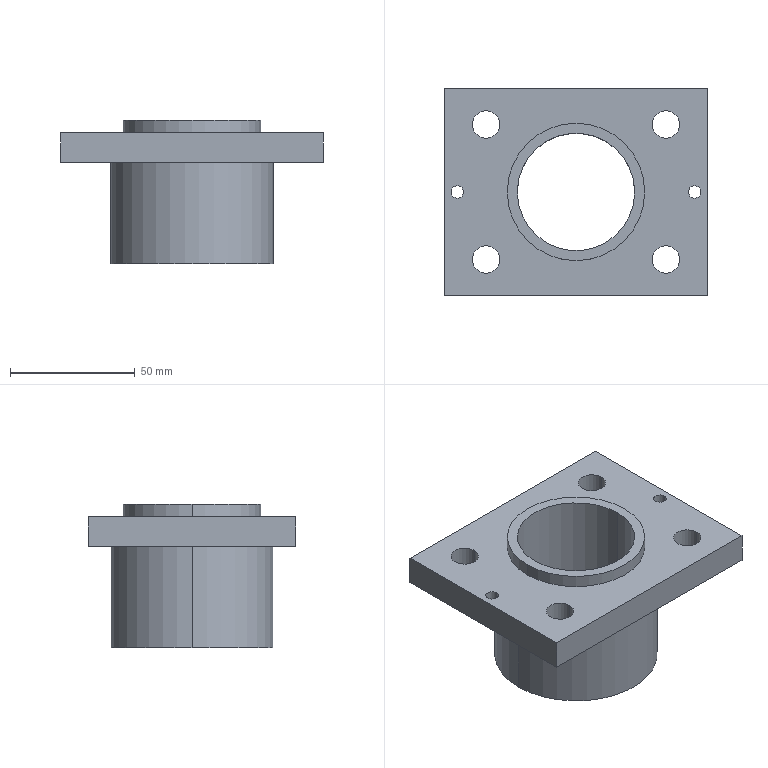Component | SolidWorks | 12AEncoderWheel-1_12AEncoderAxisRearBaffle-1 | 1 solid | 32 faces | box 105 x 83 x 57.5 mm | volume 145601 mm3 | cylinder 22 | plane 10 | commonest cylinder face diameters 11 x8 5 x4 47 x4 50 x2 55 x2 65 x2
build123d program:
from build123d import *

# Parameters (mm, degrees)
SKETCH1_W           = 83
SKETCH1_H           = 105
BOSS_EXTRUDE1_DEPTH = 12
SKETCH2_R           = 32.5
BOSS_EXTRUDE2_DEPTH = 57.5
SKETCH3_R           = 32.5
SKETCH3_R_2         = 27.5
CUT_EXTRUDE1_DEPTH  = 5
SKETCH4_R           = 23.5
CUT_EXTRUDE2_DEPTH  = 89.231
CUT_EXTRUDE5_REACH  = 87.057
SKETCH7_R           = 5.5
M6_TAPPED_HOLE1_D   = 5
SKETCH10_W          = 25
SKETCH10_H          = 2


with BuildPart() as part:
    # Sketch1 → Boss-Extrude1 (new body)
    with BuildSketch(Plane(origin=(0, 0, 0), x_dir=(1, 0, 0), z_dir=(0, 1, 0))):
        Rectangle(SKETCH1_W, SKETCH1_H)
    extrude(amount=BOSS_EXTRUDE1_DEPTH)

    # Sketch2 → Boss-Extrude2 (add)
    with BuildSketch(Plane.XZ.offset(5)):
        with Locations(Location((0, 0, 0), (0, 0, 270))):
            Circle(SKETCH2_R)
    extrude(amount=-BOSS_EXTRUDE2_DEPTH)

    # Sketch3 → Cut-Extrude1 (cut)
    with BuildSketch(Plane.XZ.offset(5)):
        with Locations(Location((0, 0, 0), (0, 0, 270))):
            Circle(SKETCH3_R)
        with Locations(Location((0, 0, 0), (0, 0, 270))):
            Circle(SKETCH3_R_2, mode=Mode.SUBTRACT)
    extrude(amount=-CUT_EXTRUDE1_DEPTH, mode=Mode.SUBTRACT)

    # Sketch4 → Cut-Extrude2 (cut, through all)
    with BuildSketch(Plane(origin=(0, 52.5, 0), x_dir=(1, 0, 0), z_dir=(0, 1, 0))):
        with Locations(Location((0, 0, 0), (0, 0, 270))):
            Circle(SKETCH4_R)
    extrude(amount=-CUT_EXTRUDE2_DEPTH, mode=Mode.SUBTRACT)

    # Sketch7 → Cut-Extrude5 (cut, up to next)
    with BuildSketch(Plane.XZ, mode=Mode.PRIVATE) as cut_extrude5_sk1:
        with Locations(Location((-27, 36, 0), (0, 0, 270))):
            Circle(SKETCH7_R)
    cut_extrude5_tool1 = extrude(cut_extrude5_sk1.sketch, amount=-CUT_EXTRUDE5_REACH, mode=Mode.PRIVATE) & part.part
    # Sketch7 → Cut-Extrude5 (cut, up to next)
    with BuildSketch(Plane.XZ, mode=Mode.PRIVATE) as cut_extrude5_sk2:
        with Locations(Location((27, 36, 0), (0, 0, 90))):
            Circle(SKETCH7_R)
    cut_extrude5_tool2 = extrude(cut_extrude5_sk2.sketch, amount=-CUT_EXTRUDE5_REACH, mode=Mode.PRIVATE) & part.part
    # Sketch7 → Cut-Extrude5 (cut, up to next)
    with BuildSketch(Plane.XZ, mode=Mode.PRIVATE) as cut_extrude5_sk3:
        with Locations(Location((27, -36, 0), (0, 0, 270))):
            Circle(SKETCH7_R)
    cut_extrude5_tool3 = extrude(cut_extrude5_sk3.sketch, amount=-CUT_EXTRUDE5_REACH, mode=Mode.PRIVATE) & part.part
    # Sketch7 → Cut-Extrude5 (cut, up to next)
    with BuildSketch(Plane.XZ, mode=Mode.PRIVATE) as cut_extrude5_sk4:
        with Locations(Location((-27, -36, 0), (0, 0, 90))):
            Circle(SKETCH7_R)
    cut_extrude5_tool4 = extrude(cut_extrude5_sk4.sketch, amount=-CUT_EXTRUDE5_REACH, mode=Mode.PRIVATE) & part.part
    add(cut_extrude5_tool1.solids().sort_by_distance((-27, 0, 36))[0], mode=Mode.SUBTRACT)
    add(cut_extrude5_tool2.solids().sort_by_distance((27, 0, 36))[0], mode=Mode.SUBTRACT)
    add(cut_extrude5_tool3.solids().sort_by_distance((27, 0, -36))[0], mode=Mode.SUBTRACT)
    add(cut_extrude5_tool4.solids().sort_by_distance((-27, 0, -36))[0], mode=Mode.SUBTRACT)

    # M6 Tapped Hole1 (through all)
    with Locations(Plane(origin=(0, 12, 0), x_dir=(1, 0, 0), z_dir=(0, 1, 0))):
        with Locations((0, 47.5), (0, -47.5)):
            Hole(M6_TAPPED_HOLE1_D / 2)

    # Sketch10 → Cut-Revolve1 (revolve, cut)
    with BuildSketch(Plane.XY, mode=Mode.PRIVATE) as cut_revolve1_sk:
        with Locations((12.5, 48.5)):
            Rectangle(SKETCH10_W, SKETCH10_H)
    revolve(cut_revolve1_sk.sketch.rotate(Axis((0, 0, 0), (0, 1, 0)), 270), axis=Axis((0, 0, 0), (0, 1, 0)), mode=Mode.SUBTRACT)


solid = part.part

# Placed as in the assembly
solid = solid.moved(Location((120.894, 147.181, -14.25), (-90, 90, 0)))
STEP:
#1=COLOUR_RGB('',0.7922,0.8196,0.9333);
#2=FILL_AREA_STYLE_COLOUR('',#1);
#3=FILL_AREA_STYLE('',(#2));
#4=SURFACE_STYLE_FILL_AREA(#3);
#5=SURFACE_SIDE_STYLE('',(#4));
#6=SURFACE_STYLE_USAGE(.BOTH.,#5);
#7=PRESENTATION_STYLE_ASSIGNMENT((#6));
#8=CARTESIAN_POINT('',(5.744,5.795,-2.51));
#9=VERTEX_POINT('',#8);
#10=CARTESIAN_POINT('',(3.775,5.795,-2.51));
#11=VERTEX_POINT('',#10);
#12=CARTESIAN_POINT('',(4.76,5.795,-2.51));
#13=DIRECTION('',(0.,0.,1.));
#14=DIRECTION('',(-1.,0.,0.));
#15=AXIS2_PLACEMENT_3D('',#12,#13,#14);
#16=CIRCLE('',#15,0.9843);
#17=EDGE_CURVE('',#9,#11,#16,.T.);
#18=ORIENTED_EDGE('',*,*,#17,.F.);
#19=CARTESIAN_POINT('',(5.744,5.795,-2.431));
#20=VERTEX_POINT('',#19);
#21=CARTESIAN_POINT('',(5.744,5.795,-0.561));
#22=DIRECTION('',(0.,0.,1.));
#23=VECTOR('',#22,39.37);
#24=LINE('',#21,#23);
#25=EDGE_CURVE('',#9,#20,#24,.T.);
#26=ORIENTED_EDGE('',*,*,#25,.T.);
#27=CARTESIAN_POINT('',(3.775,5.795,-2.431));
#28=VERTEX_POINT('',#27);
#29=CARTESIAN_POINT('',(4.76,5.795,-2.431));
#30=DIRECTION('',(0.,0.,1.));
#31=DIRECTION('',(-1.,0.,0.));
#32=AXIS2_PLACEMENT_3D('',#29,#30,#31);
#33=CIRCLE('',#32,0.9843);
#34=EDGE_CURVE('',#20,#28,#33,.T.);
#35=ORIENTED_EDGE('',*,*,#34,.T.);
#36=CARTESIAN_POINT('',(3.775,5.795,-0.561));
#37=DIRECTION('',(0.,0.,1.));
#38=VECTOR('',#37,39.37);
#39=LINE('',#36,#38);
#40=EDGE_CURVE('',#11,#28,#39,.T.);
#41=ORIENTED_EDGE('',*,*,#40,.F.);
#42=EDGE_LOOP('',(#18,#26,#35,#41));
#43=FACE_OUTER_BOUND('',#42,.T.);
#44=CARTESIAN_POINT('',(4.76,5.795,-0.561));
#45=DIRECTION('',(0.,0.,1.));
#46=DIRECTION('',(-1.,0.,0.));
#47=AXIS2_PLACEMENT_3D('',#44,#45,#46);
#48=CYLINDRICAL_SURFACE('',#47,0.9843);
#49=ADVANCED_FACE('',(#43),#48,.F.);
#50=CARTESIAN_POINT('',(2.791,5.795,-0.561));
#51=VERTEX_POINT('',#50);
#52=CARTESIAN_POINT('',(2.988,5.795,-0.561));
#53=VERTEX_POINT('',#52);
#54=CARTESIAN_POINT('',(2.89,5.795,-0.561));
#55=DIRECTION('',(-0.,-0.,-1.));
#56=DIRECTION('',(1.,0.,0.));
#57=AXIS2_PLACEMENT_3D('',#54,#55,#56);
#58=CIRCLE('',#57,0.09843);
#59=EDGE_CURVE('',#51,#53,#58,.T.);
#60=ORIENTED_EDGE('',*,*,#59,.F.);
#61=CARTESIAN_POINT('',(2.791,5.795,-1.033));
#62=VERTEX_POINT('',#61);
#63=CARTESIAN_POINT('',(2.791,5.795,-1.033));
#64=DIRECTION('',(-0.,-0.,-1.));
#65=VECTOR('',#64,39.37);
#66=LINE('',#63,#65);
#67=EDGE_CURVE('',#51,#62,#66,.T.);
#68=ORIENTED_EDGE('',*,*,#67,.T.);
#69=CARTESIAN_POINT('',(2.988,5.795,-1.033));
#70=VERTEX_POINT('',#69);
#71=CARTESIAN_POINT('',(2.89,5.795,-1.033));
#72=DIRECTION('',(-0.,-0.,-1.));
#73=DIRECTION('',(1.,0.,0.));
#74=AXIS2_PLACEMENT_3D('',#71,#72,#73);
#75=CIRCLE('',#74,0.09843);
#76=EDGE_CURVE('',#62,#70,#75,.T.);
#77=ORIENTED_EDGE('',*,*,#76,.T.);
#78=CARTESIAN_POINT('',(2.988,5.795,-1.033));
#79=DIRECTION('',(-0.,-0.,-1.));
#80=VECTOR('',#79,39.37);
#81=LINE('',#78,#80);
#82=EDGE_CURVE('',#53,#70,#81,.T.);
#83=ORIENTED_EDGE('',*,*,#82,.F.);
#84=EDGE_LOOP('',(#60,#68,#77,#83));
#85=FACE_OUTER_BOUND('',#84,.T.);
#86=CARTESIAN_POINT('',(2.89,5.795,-1.033));
#87=DIRECTION('',(-0.,-0.,-1.));
#88=DIRECTION('',(1.,0.,0.));
#89=AXIS2_PLACEMENT_3D('',#86,#87,#88);
#90=CYLINDRICAL_SURFACE('',#89,0.09843);
#91=ADVANCED_FACE('',(#85),#90,.F.);
#92=CARTESIAN_POINT('',(6.531,5.795,-0.561));
#93=VERTEX_POINT('',#92);
#94=CARTESIAN_POINT('',(6.728,5.795,-0.561));
#95=VERTEX_POINT('',#94);
#96=CARTESIAN_POINT('',(6.63,5.795,-0.561));
#97=DIRECTION('',(-0.,-0.,-1.));
#98=DIRECTION('',(1.,0.,0.));
#99=AXIS2_PLACEMENT_3D('',#96,#97,#98);
#100=CIRCLE('',#99,0.09843);
#101=EDGE_CURVE('',#93,#95,#100,.T.);
#102=ORIENTED_EDGE('',*,*,#101,.F.);
#103=CARTESIAN_POINT('',(6.531,5.795,-1.033));
#104=VERTEX_POINT('',#103);
#105=CARTESIAN_POINT('',(6.531,5.795,-1.033));
#106=DIRECTION('',(-0.,-0.,-1.));
#107=VECTOR('',#106,39.37);
#108=LINE('',#105,#107);
#109=EDGE_CURVE('',#93,#104,#108,.T.);
#110=ORIENTED_EDGE('',*,*,#109,.T.);
#111=CARTESIAN_POINT('',(6.728,5.795,-1.033));
#112=VERTEX_POINT('',#111);
#113=CARTESIAN_POINT('',(6.63,5.795,-1.033));
#114=DIRECTION('',(-0.,-0.,-1.));
#115=DIRECTION('',(1.,0.,0.));
#116=AXIS2_PLACEMENT_3D('',#113,#114,#115);
#117=CIRCLE('',#116,0.09843);
#118=EDGE_CURVE('',#104,#112,#117,.T.);
#119=ORIENTED_EDGE('',*,*,#118,.T.);
#120=CARTESIAN_POINT('',(6.728,5.795,-1.033));
#121=DIRECTION('',(-0.,-0.,-1.));
#122=VECTOR('',#121,39.37);
#123=LINE('',#120,#122);
#124=EDGE_CURVE('',#95,#112,#123,.T.);
#125=ORIENTED_EDGE('',*,*,#124,.F.);
#126=EDGE_LOOP('',(#102,#110,#119,#125));
#127=FACE_OUTER_BOUND('',#126,.T.);
#128=CARTESIAN_POINT('',(6.63,5.795,-1.033));
#129=DIRECTION('',(-0.,-0.,-1.));
#130=DIRECTION('',(1.,0.,0.));
#131=AXIS2_PLACEMENT_3D('',#128,#129,#130);
#132=CYLINDRICAL_SURFACE('',#131,0.09843);
#133=ADVANCED_FACE('',(#127),#132,.F.);
#134=CARTESIAN_POINT('',(3.559,6.858,-1.033));
#135=VERTEX_POINT('',#134);
#136=CARTESIAN_POINT('',(3.126,6.858,-1.033));
#137=VERTEX_POINT('',#136);
#138=CARTESIAN_POINT('',(3.342,6.858,-1.033));
#139=DIRECTION('',(0.,0.,1.));
#140=DIRECTION('',(1.,0.,0.));
#141=AXIS2_PLACEMENT_3D('',#138,#139,#140);
#142=CIRCLE('',#141,0.2165);
#143=EDGE_CURVE('',#135,#137,#142,.T.);
#144=ORIENTED_EDGE('',*,*,#143,.F.);
#145=CARTESIAN_POINT('',(3.559,6.858,-0.561));
#146=VERTEX_POINT('',#145);
#147=CARTESIAN_POINT('',(3.559,6.858,-2.628));
#148=DIRECTION('',(0.,0.,1.));
#149=VECTOR('',#148,39.37);
#150=LINE('',#147,#149);
#151=EDGE_CURVE('',#135,#146,#150,.T.);
#152=ORIENTED_EDGE('',*,*,#151,.T.);
#153=CARTESIAN_POINT('',(3.126,6.858,-0.561));
#154=VERTEX_POINT('',#153);
#155=CARTESIAN_POINT('',(3.342,6.858,-0.561));
#156=DIRECTION('',(0.,0.,1.));
#157=DIRECTION('',(1.,0.,0.));
#158=AXIS2_PLACEMENT_3D('',#155,#156,#157);
#159=CIRCLE('',#158,0.2165);
#160=EDGE_CURVE('',#146,#154,#159,.T.);
#161=ORIENTED_EDGE('',*,*,#160,.T.);
#162=CARTESIAN_POINT('',(3.126,6.858,-2.628));
#163=DIRECTION('',(0.,0.,1.));
#164=VECTOR('',#163,39.37);
#165=LINE('',#162,#164);
#166=EDGE_CURVE('',#137,#154,#165,.T.);
#167=ORIENTED_EDGE('',*,*,#166,.F.);
#168=EDGE_LOOP('',(#144,#152,#161,#167));
#169=FACE_OUTER_BOUND('',#168,.T.);
#170=CARTESIAN_POINT('',(3.342,6.858,-2.628));
#171=DIRECTION('',(0.,0.,1.));
#172=DIRECTION('',(-1.,0.,0.));
#173=AXIS2_PLACEMENT_3D('',#170,#171,#172);
#174=CYLINDRICAL_SURFACE('',#173,0.2165);
#175=ADVANCED_FACE('',(#169),#174,.F.);
#176=CARTESIAN_POINT('',(3.559,4.732,-1.033));
#177=VERTEX_POINT('',#176);
#178=CARTESIAN_POINT('',(3.126,4.732,-1.033));
#179=VERTEX_POINT('',#178);
#180=CARTESIAN_POINT('',(3.342,4.732,-1.033));
#181=DIRECTION('',(0.,0.,1.));
#182=DIRECTION('',(1.,0.,0.));
#183=AXIS2_PLACEMENT_3D('',#180,#181,#182);
#184=CIRCLE('',#183,0.2165);
#185=EDGE_CURVE('',#177,#179,#184,.T.);
#186=ORIENTED_EDGE('',*,*,#185,.F.);
#187=CARTESIAN_POINT('',(3.559,4.732,-0.561));
#188=VERTEX_POINT('',#187);
#189=CARTESIAN_POINT('',(3.559,4.732,-2.628));
#190=DIRECTION('',(0.,0.,1.));
#191=VECTOR('',#190,39.37);
#192=LINE('',#189,#191);
#193=EDGE_CURVE('',#177,#188,#192,.T.);
#194=ORIENTED_EDGE('',*,*,#193,.T.);
#195=CARTESIAN_POINT('',(3.126,4.732,-0.561));
#196=VERTEX_POINT('',#195);
#197=CARTESIAN_POINT('',(3.342,4.732,-0.561));
#198=DIRECTION('',(0.,0.,1.));
#199=DIRECTION('',(-1.,0.,0.));
#200=AXIS2_PLACEMENT_3D('',#197,#198,#199);
#201=CIRCLE('',#200,0.2165);
#202=EDGE_CURVE('',#188,#196,#201,.T.);
#203=ORIENTED_EDGE('',*,*,#202,.T.);
#204=CARTESIAN_POINT('',(3.126,4.732,-2.628));
#205=DIRECTION('',(0.,0.,1.));
#206=VECTOR('',#205,39.37);
#207=LINE('',#204,#206);
#208=EDGE_CURVE('',#179,#196,#207,.T.);
#209=ORIENTED_EDGE('',*,*,#208,.F.);
#210=EDGE_LOOP('',(#186,#194,#203,#209));
#211=FACE_OUTER_BOUND('',#210,.T.);
#212=CARTESIAN_POINT('',(3.342,4.732,-2.628));
#213=DIRECTION('',(0.,0.,1.));
#214=DIRECTION('',(-1.,0.,0.));
#215=AXIS2_PLACEMENT_3D('',#212,#213,#214);
#216=CYLINDRICAL_SURFACE('',#215,0.2165);
#217=ADVANCED_FACE('',(#211),#216,.F.);
#218=CARTESIAN_POINT('',(6.393,4.732,-1.033));
#219=VERTEX_POINT('',#218);
#220=CARTESIAN_POINT('',(5.96,4.732,-1.033));
#221=VERTEX_POINT('',#220);
#222=CARTESIAN_POINT('',(6.177,4.732,-1.033));
#223=DIRECTION('',(0.,0.,1.));
#224=DIRECTION('',(1.,0.,0.));
#225=AXIS2_PLACEMENT_3D('',#222,#223,#224);
#226=CIRCLE('',#225,0.2165);
#227=EDGE_CURVE('',#219,#221,#226,.T.);
#228=ORIENTED_EDGE('',*,*,#227,.F.);
#229=CARTESIAN_POINT('',(6.393,4.732,-0.561));
#230=VERTEX_POINT('',#229);
#231=CARTESIAN_POINT('',(6.393,4.732,-2.628));
#232=DIRECTION('',(0.,0.,1.));
#233=VECTOR('',#232,39.37);
#234=LINE('',#231,#233);
#235=EDGE_CURVE('',#219,#230,#234,.T.);
#236=ORIENTED_EDGE('',*,*,#235,.T.);
#237=CARTESIAN_POINT('',(5.96,4.732,-0.561));
#238=VERTEX_POINT('',#237);
#239=CARTESIAN_POINT('',(6.177,4.732,-0.561));
#240=DIRECTION('',(0.,0.,1.));
#241=DIRECTION('',(1.,0.,0.));
#242=AXIS2_PLACEMENT_3D('',#239,#240,#241);
#243=CIRCLE('',#242,0.2165);
#244=EDGE_CURVE('',#230,#238,#243,.T.);
#245=ORIENTED_EDGE('',*,*,#244,.T.);
#246=CARTESIAN_POINT('',(5.96,4.732,-2.628));
#247=DIRECTION('',(0.,0.,1.));
#248=VECTOR('',#247,39.37);
#249=LINE('',#246,#248);
#250=EDGE_CURVE('',#221,#238,#249,.T.);
#251=ORIENTED_EDGE('',*,*,#250,.F.);
#252=EDGE_LOOP('',(#228,#236,#245,#251));
#253=FACE_OUTER_BOUND('',#252,.T.);
#254=CARTESIAN_POINT('',(6.177,4.732,-2.628));
#255=DIRECTION('',(0.,0.,1.));
#256=DIRECTION('',(-1.,0.,0.));
#257=AXIS2_PLACEMENT_3D('',#254,#255,#256);
#258=CYLINDRICAL_SURFACE('',#257,0.2165);
#259=ADVANCED_FACE('',(#253),#258,.F.);
#260=CARTESIAN_POINT('',(6.393,6.858,-1.033));
#261=VERTEX_POINT('',#260);
#262=CARTESIAN_POINT('',(5.96,6.858,-1.033));
#263=VERTEX_POINT('',#262);
#264=CARTESIAN_POINT('',(6.177,6.858,-1.033));
#265=DIRECTION('',(0.,0.,1.));
#266=DIRECTION('',(1.,0.,0.));
#267=AXIS2_PLACEMENT_3D('',#264,#265,#266);
#268=CIRCLE('',#267,0.2165);
#269=EDGE_CURVE('',#261,#263,#268,.T.);
#270=ORIENTED_EDGE('',*,*,#269,.F.);
#271=CARTESIAN_POINT('',(6.393,6.858,-0.561));
#272=VERTEX_POINT('',#271);
#273=CARTESIAN_POINT('',(6.393,6.858,-2.628));
#274=DIRECTION('',(0.,0.,1.));
#275=VECTOR('',#274,39.37);
#276=LINE('',#273,#275);
#277=EDGE_CURVE('',#261,#272,#276,.T.);
#278=ORIENTED_EDGE('',*,*,#277,.T.);
#279=CARTESIAN_POINT('',(5.96,6.858,-0.561));
#280=VERTEX_POINT('',#279);
#281=CARTESIAN_POINT('',(6.177,6.858,-0.561));
#282=DIRECTION('',(0.,0.,1.));
#283=DIRECTION('',(-1.,0.,0.));
#284=AXIS2_PLACEMENT_3D('',#281,#282,#283);
#285=CIRCLE('',#284,0.2165);
#286=EDGE_CURVE('',#272,#280,#285,.T.);
#287=ORIENTED_EDGE('',*,*,#286,.T.);
#288=CARTESIAN_POINT('',(5.96,6.858,-2.628));
#289=DIRECTION('',(0.,0.,1.));
#290=VECTOR('',#289,39.37);
#291=LINE('',#288,#290);
#292=EDGE_CURVE('',#263,#280,#291,.T.);
#293=ORIENTED_EDGE('',*,*,#292,.F.);
#294=EDGE_LOOP('',(#270,#278,#287,#293));
#295=FACE_OUTER_BOUND('',#294,.T.);
#296=CARTESIAN_POINT('',(6.177,6.858,-2.628));
#297=DIRECTION('',(0.,0.,1.));
#298=DIRECTION('',(-1.,0.,0.));
#299=AXIS2_PLACEMENT_3D('',#296,#297,#298);
#300=CYLINDRICAL_SURFACE('',#299,0.2165);
#301=ADVANCED_FACE('',(#295),#300,.F.);
#302=CARTESIAN_POINT('',(3.834,5.795,-0.3642));
#303=VERTEX_POINT('',#302);
#304=CARTESIAN_POINT('',(5.685,5.795,-0.3642));
#305=VERTEX_POINT('',#304);
#306=CARTESIAN_POINT('',(4.76,5.795,-0.3642));
#307=DIRECTION('',(-0.,-0.,-1.));
#308=DIRECTION('',(1.,0.,0.));
#309=AXIS2_PLACEMENT_3D('',#306,#307,#308);
#310=CIRCLE('',#309,0.9252);
#311=EDGE_CURVE('',#303,#305,#310,.T.);
#312=ORIENTED_EDGE('',*,*,#311,.F.);
#313=CARTESIAN_POINT('',(3.834,5.795,-2.431));
#314=VERTEX_POINT('',#313);
#315=CARTESIAN_POINT('',(3.834,5.795,-0.3642));
#316=DIRECTION('',(-0.,-0.,-1.));
#317=VECTOR('',#316,39.37);
#318=LINE('',#315,#317);
#319=EDGE_CURVE('',#303,#314,#318,.T.);
#320=ORIENTED_EDGE('',*,*,#319,.T.);
#321=CARTESIAN_POINT('',(5.685,5.795,-2.431));
#322=VERTEX_POINT('',#321);
#323=CARTESIAN_POINT('',(4.76,5.795,-2.431));
#324=DIRECTION('',(-0.,-0.,-1.));
#325=DIRECTION('',(-1.,0.,0.));
#326=AXIS2_PLACEMENT_3D('',#323,#324,#325);
#327=CIRCLE('',#326,0.9252);
#328=EDGE_CURVE('',#314,#322,#327,.T.);
#329=ORIENTED_EDGE('',*,*,#328,.T.);
#330=CARTESIAN_POINT('',(5.685,5.795,-0.3642));
#331=DIRECTION('',(-0.,-0.,-1.));
#332=VECTOR('',#331,39.37);
#333=LINE('',#330,#332);
#334=EDGE_CURVE('',#305,#322,#333,.T.);
#335=ORIENTED_EDGE('',*,*,#334,.F.);
#336=EDGE_LOOP('',(#312,#320,#329,#335));
#337=FACE_OUTER_BOUND('',#336,.T.);
#338=CARTESIAN_POINT('',(4.76,5.795,-0.3642));
#339=DIRECTION('',(-0.,-0.,-1.));
#340=DIRECTION('',(1.,0.,0.));
#341=AXIS2_PLACEMENT_3D('',#338,#339,#340);
#342=CYLINDRICAL_SURFACE('',#341,0.9252);
#343=ADVANCED_FACE('',(#337),#342,.F.);
#344=CARTESIAN_POINT('',(3.677,5.795,-0.561));
#345=VERTEX_POINT('',#344);
#346=CARTESIAN_POINT('',(5.842,5.795,-0.561));
#347=VERTEX_POINT('',#346);
#348=CARTESIAN_POINT('',(4.76,5.795,-0.561));
#349=DIRECTION('',(0.,0.,1.));
#350=DIRECTION('',(-1.,0.,0.));
#351=AXIS2_PLACEMENT_3D('',#348,#349,#350);
#352=CIRCLE('',#351,1.083);
#353=EDGE_CURVE('',#345,#347,#352,.T.);
#354=ORIENTED_EDGE('',*,*,#353,.T.);
#355=CARTESIAN_POINT('',(5.842,5.795,-0.3642));
#356=VERTEX_POINT('',#355);
#357=CARTESIAN_POINT('',(5.842,5.795,-0.561));
#358=DIRECTION('',(0.,0.,1.));
#359=VECTOR('',#358,39.37);
#360=LINE('',#357,#359);
#361=EDGE_CURVE('',#347,#356,#360,.T.);
#362=ORIENTED_EDGE('',*,*,#361,.T.);
#363=CARTESIAN_POINT('',(3.677,5.795,-0.3642));
#364=VERTEX_POINT('',#363);
#365=CARTESIAN_POINT('',(4.76,5.795,-0.3642));
#366=DIRECTION('',(0.,0.,1.));
#367=DIRECTION('',(-1.,0.,0.));
#368=AXIS2_PLACEMENT_3D('',#365,#366,#367);
#369=CIRCLE('',#368,1.083);
#370=EDGE_CURVE('',#364,#356,#369,.T.);
#371=ORIENTED_EDGE('',*,*,#370,.F.);
#372=CARTESIAN_POINT('',(3.677,5.795,-0.561));
#373=DIRECTION('',(0.,0.,1.));
#374=VECTOR('',#373,39.37);
#375=LINE('',#372,#374);
#376=EDGE_CURVE('',#345,#364,#375,.T.);
#377=ORIENTED_EDGE('',*,*,#376,.F.);
#378=EDGE_LOOP('',(#354,#362,#371,#377));
#379=FACE_OUTER_BOUND('',#378,.T.);
#380=CARTESIAN_POINT('',(4.76,5.795,-0.561));
#381=DIRECTION('',(0.,0.,1.));
#382=DIRECTION('',(-1.,0.,0.));
#383=AXIS2_PLACEMENT_3D('',#380,#381,#382);
#384=CYLINDRICAL_SURFACE('',#383,1.083);
#385=ADVANCED_FACE('',(#379),#384,.T.);
#386=CARTESIAN_POINT('',(3.48,5.795,-2.628));
#387=VERTEX_POINT('',#386);
#388=CARTESIAN_POINT('',(6.039,5.795,-2.628));
#389=VERTEX_POINT('',#388);
#390=CARTESIAN_POINT('',(4.76,5.795,-2.628));
#391=DIRECTION('',(0.,0.,1.));
#392=DIRECTION('',(-1.,0.,0.));
#393=AXIS2_PLACEMENT_3D('',#390,#391,#392);
#394=CIRCLE('',#393,1.28);
#395=EDGE_CURVE('',#387,#389,#394,.T.);
#396=ORIENTED_EDGE('',*,*,#395,.T.);
#397=CARTESIAN_POINT('',(6.039,5.795,-1.033));
#398=VERTEX_POINT('',#397);
#399=CARTESIAN_POINT('',(6.039,5.795,-2.628));
#400=DIRECTION('',(0.,0.,1.));
#401=VECTOR('',#400,39.37);
#402=LINE('',#399,#401);
#403=EDGE_CURVE('',#389,#398,#402,.T.);
#404=ORIENTED_EDGE('',*,*,#403,.T.);
#405=CARTESIAN_POINT('',(3.48,5.795,-1.033));
#406=VERTEX_POINT('',#405);
#407=CARTESIAN_POINT('',(4.76,5.795,-1.033));
#408=DIRECTION('',(-0.,-0.,-1.));
#409=DIRECTION('',(1.,0.,0.));
#410=AXIS2_PLACEMENT_3D('',#407,#408,#409);
#411=CIRCLE('',#410,1.28);
#412=EDGE_CURVE('',#398,#406,#411,.T.);
#413=ORIENTED_EDGE('',*,*,#412,.T.);
#414=CARTESIAN_POINT('',(3.48,5.795,-2.628));
#415=DIRECTION('',(0.,0.,1.));
#416=VECTOR('',#415,39.37);
#417=LINE('',#414,#416);
#418=EDGE_CURVE('',#387,#406,#417,.T.);
#419=ORIENTED_EDGE('',*,*,#418,.F.);
#420=EDGE_LOOP('',(#396,#404,#413,#419));
#421=FACE_OUTER_BOUND('',#420,.T.);
#422=CARTESIAN_POINT('',(4.76,5.795,-2.628));
#423=DIRECTION('',(0.,0.,1.));
#424=DIRECTION('',(-1.,0.,0.));
#425=AXIS2_PLACEMENT_3D('',#422,#423,#424);
#426=CYLINDRICAL_SURFACE('',#425,1.28);
#427=ADVANCED_FACE('',(#421),#426,.T.);
#428=CARTESIAN_POINT('',(5.685,5.795,-2.51));
#429=VERTEX_POINT('',#428);
#430=CARTESIAN_POINT('',(3.834,5.795,-2.51));
#431=VERTEX_POINT('',#430);
#432=CARTESIAN_POINT('',(4.76,5.795,-2.51));
#433=DIRECTION('',(0.,0.,1.));
#434=DIRECTION('',(1.,0.,0.));
#435=AXIS2_PLACEMENT_3D('',#432,#433,#434);
#436=CIRCLE('',#435,0.9252);
#437=EDGE_CURVE('',#429,#431,#436,.T.);
#438=ORIENTED_EDGE('',*,*,#437,.T.);
#439=CARTESIAN_POINT('',(3.834,5.795,-2.628));
#440=VERTEX_POINT('',#439);
#441=CARTESIAN_POINT('',(3.834,5.795,-0.3642));
#442=DIRECTION('',(-0.,-0.,-1.));
#443=VECTOR('',#442,39.37);
#444=LINE('',#441,#443);
#445=EDGE_CURVE('',#431,#440,#444,.T.);
#446=ORIENTED_EDGE('',*,*,#445,.T.);
#447=CARTESIAN_POINT('',(5.685,5.795,-2.628));
#448=VERTEX_POINT('',#447);
#449=CARTESIAN_POINT('',(4.76,5.795,-2.628));
#450=DIRECTION('',(-0.,-0.,-1.));
#451=DIRECTION('',(1.,0.,0.));
#452=AXIS2_PLACEMENT_3D('',#449,#450,#451);
#453=CIRCLE('',#452,0.9252);
#454=EDGE_CURVE('',#440,#448,#453,.T.);
#455=ORIENTED_EDGE('',*,*,#454,.T.);
#456=CARTESIAN_POINT('',(5.685,5.795,-0.3642));
#457=DIRECTION('',(-0.,-0.,-1.));
#458=VECTOR('',#457,39.37);
#459=LINE('',#456,#458);
#460=EDGE_CURVE('',#429,#448,#459,.T.);
#461=ORIENTED_EDGE('',*,*,#460,.F.);
#462=EDGE_LOOP('',(#438,#446,#455,#461));
#463=FACE_OUTER_BOUND('',#462,.T.);
#464=CARTESIAN_POINT('',(4.76,5.795,-0.3642));
#465=DIRECTION('',(-0.,-0.,-1.));
#466=DIRECTION('',(1.,0.,0.));
#467=AXIS2_PLACEMENT_3D('',#464,#465,#466);
#468=CYLINDRICAL_SURFACE('',#467,0.9252);
#469=ADVANCED_FACE('',(#463),#468,.F.);
#470=ORIENTED_EDGE('',*,*,#445,.F.);
#471=CARTESIAN_POINT('',(4.76,5.795,-2.51));
#472=DIRECTION('',(0.,0.,1.));
#473=DIRECTION('',(1.,0.,0.));
#474=AXIS2_PLACEMENT_3D('',#471,#472,#473);
#475=CIRCLE('',#474,0.9252);
#476=EDGE_CURVE('',#431,#429,#475,.T.);
#477=ORIENTED_EDGE('',*,*,#476,.T.);
#478=ORIENTED_EDGE('',*,*,#460,.T.);
#479=CARTESIAN_POINT('',(4.76,5.795,-2.628));
#480=DIRECTION('',(-0.,-0.,-1.));
#481=DIRECTION('',(1.,0.,0.));
#482=AXIS2_PLACEMENT_3D('',#479,#480,#481);
#483=CIRCLE('',#482,0.9252);
#484=EDGE_CURVE('',#448,#440,#483,.T.);
#485=ORIENTED_EDGE('',*,*,#484,.T.);
#486=EDGE_LOOP('',(#470,#477,#478,#485));
#487=FACE_OUTER_BOUND('',#486,.T.);
#488=CARTESIAN_POINT('',(4.76,5.795,-0.3642));
#489=DIRECTION('',(-0.,-0.,-1.));
#490=DIRECTION('',(1.,0.,0.));
#491=AXIS2_PLACEMENT_3D('',#488,#489,#490);
#492=CYLINDRICAL_SURFACE('',#491,0.9252);
#493=ADVANCED_FACE('',(#487),#492,.F.);
#494=CARTESIAN_POINT('',(6.827,4.161,-0.561));
#495=VERTEX_POINT('',#494);
#496=CARTESIAN_POINT('',(2.693,4.161,-0.561));
#497=VERTEX_POINT('',#496);
#498=CARTESIAN_POINT('',(2.693,4.161,-0.561));
#499=DIRECTION('',(-1.,-0.,0.));
#500=VECTOR('',#499,39.37);
#501=LINE('',#498,#500);
#502=EDGE_CURVE('',#495,#497,#501,.T.);
#503=ORIENTED_EDGE('',*,*,#502,.T.);
#504=CARTESIAN_POINT('',(2.693,4.161,-1.033));
#505=VERTEX_POINT('',#504);
#506=CARTESIAN_POINT('',(2.693,4.161,-1.033));
#507=DIRECTION('',(0.,0.,1.));
#508=VECTOR('',#507,39.37);
#509=LINE('',#506,#508);
#510=EDGE_CURVE('',#505,#497,#509,.T.);
#511=ORIENTED_EDGE('',*,*,#510,.F.);
#512=CARTESIAN_POINT('',(6.827,4.161,-1.033));
#513=VERTEX_POINT('',#512);
#514=CARTESIAN_POINT('',(2.693,4.161,-1.033));
#515=DIRECTION('',(-1.,-0.,0.));
#516=VECTOR('',#515,39.37);
#517=LINE('',#514,#516);
#518=EDGE_CURVE('',#513,#505,#517,.T.);
#519=ORIENTED_EDGE('',*,*,#518,.F.);
#520=CARTESIAN_POINT('',(6.827,4.161,-1.033));
#521=DIRECTION('',(0.,0.,1.));
#522=VECTOR('',#521,39.37);
#523=LINE('',#520,#522);
#524=EDGE_CURVE('',#513,#495,#523,.T.);
#525=ORIENTED_EDGE('',*,*,#524,.T.);
#526=EDGE_LOOP('',(#503,#511,#519,#525));
#527=FACE_OUTER_BOUND('',#526,.T.);
#528=CARTESIAN_POINT('',(2.693,4.161,-1.033));
#529=DIRECTION('',(-0.,1.,-0.));
#530=DIRECTION('',(1.,0.,-0.));
#531=AXIS2_PLACEMENT_3D('',#528,#529,#530);
#532=PLANE('',#531);
#533=ADVANCED_FACE('',(#527),#532,.F.);
#534=CARTESIAN_POINT('',(2.693,7.428,-0.561));
#535=VERTEX_POINT('',#534);
#536=CARTESIAN_POINT('',(2.693,7.428,-0.561));
#537=DIRECTION('',(-0.,1.,-0.));
#538=VECTOR('',#537,39.37);
#539=LINE('',#536,#538);
#540=EDGE_CURVE('',#497,#535,#539,.T.);
#541=ORIENTED_EDGE('',*,*,#540,.T.);
#542=CARTESIAN_POINT('',(2.693,7.428,-1.033));
#543=VERTEX_POINT('',#542);
#544=CARTESIAN_POINT('',(2.693,7.428,-1.033));
#545=DIRECTION('',(0.,0.,1.));
#546=VECTOR('',#545,39.37);
#547=LINE('',#544,#546);
#548=EDGE_CURVE('',#543,#535,#547,.T.);
#549=ORIENTED_EDGE('',*,*,#548,.F.);
#550=CARTESIAN_POINT('',(2.693,7.428,-1.033));
#551=DIRECTION('',(-0.,1.,-0.));
#552=VECTOR('',#551,39.37);
#553=LINE('',#550,#552);
#554=EDGE_CURVE('',#505,#543,#553,.T.);
#555=ORIENTED_EDGE('',*,*,#554,.F.);
#556=ORIENTED_EDGE('',*,*,#510,.T.);
#557=EDGE_LOOP('',(#541,#549,#555,#556));
#558=FACE_OUTER_BOUND('',#557,.T.);
#559=CARTESIAN_POINT('',(2.693,7.428,-1.033));
#560=DIRECTION('',(1.,0.,-0.));
#561=DIRECTION('',(0.,-1.,0.));
#562=AXIS2_PLACEMENT_3D('',#559,#560,#561);
#563=PLANE('',#562);
#564=ADVANCED_FACE('',(#558),#563,.F.);
#565=CARTESIAN_POINT('',(6.827,7.428,-0.561));
#566=VERTEX_POINT('',#565);
#567=CARTESIAN_POINT('',(2.693,7.428,-0.561));
#568=DIRECTION('',(1.,0.,-0.));
#569=VECTOR('',#568,39.37);
#570=LINE('',#567,#569);
#571=EDGE_CURVE('',#535,#566,#570,.T.);
#572=ORIENTED_EDGE('',*,*,#571,.T.);
#573=CARTESIAN_POINT('',(6.827,7.428,-1.033));
#574=VERTEX_POINT('',#573);
#575=CARTESIAN_POINT('',(6.827,7.428,-1.033));
#576=DIRECTION('',(0.,0.,1.));
#577=VECTOR('',#576,39.37);
#578=LINE('',#575,#577);
#579=EDGE_CURVE('',#574,#566,#578,.T.);
#580=ORIENTED_EDGE('',*,*,#579,.F.);
#581=CARTESIAN_POINT('',(2.693,7.428,-1.033));
#582=DIRECTION('',(1.,0.,-0.));
#583=VECTOR('',#582,39.37);
#584=LINE('',#581,#583);
#585=EDGE_CURVE('',#543,#574,#584,.T.);
#586=ORIENTED_EDGE('',*,*,#585,.F.);
#587=ORIENTED_EDGE('',*,*,#548,.T.);
#588=EDGE_LOOP('',(#572,#580,#586,#587));
#589=FACE_OUTER_BOUND('',#588,.T.);
#590=CARTESIAN_POINT('',(2.693,7.428,-1.033));
#591=DIRECTION('',(0.,-1.,0.));
#592=DIRECTION('',(-1.,-0.,0.));
#593=AXIS2_PLACEMENT_3D('',#590,#591,#592);
#594=PLANE('',#593);
#595=ADVANCED_FACE('',(#589),#594,.F.);
#596=CARTESIAN_POINT('',(6.827,7.428,-0.561));
#597=DIRECTION('',(0.,-1.,0.));
#598=VECTOR('',#597,39.37);
#599=LINE('',#596,#598);
#600=EDGE_CURVE('',#566,#495,#599,.T.);
#601=ORIENTED_EDGE('',*,*,#600,.T.);
#602=ORIENTED_EDGE('',*,*,#524,.F.);
#603=CARTESIAN_POINT('',(6.827,7.428,-1.033));
#604=DIRECTION('',(0.,-1.,0.));
#605=VECTOR('',#604,39.37);
#606=LINE('',#603,#605);
#607=EDGE_CURVE('',#574,#513,#606,.T.);
#608=ORIENTED_EDGE('',*,*,#607,.F.);
#609=ORIENTED_EDGE('',*,*,#579,.T.);
#610=EDGE_LOOP('',(#601,#602,#608,#609));
#611=FACE_OUTER_BOUND('',#610,.T.);
#612=CARTESIAN_POINT('',(6.827,7.428,-1.033));
#613=DIRECTION('',(-1.,-0.,0.));
#614=DIRECTION('',(-0.,1.,-0.));
#615=AXIS2_PLACEMENT_3D('',#612,#613,#614);
#616=PLANE('',#615);
#617=ADVANCED_FACE('',(#611),#616,.F.);
#618=CARTESIAN_POINT('',(2.89,5.795,-1.033));
#619=DIRECTION('',(-0.,-0.,-1.));
#620=DIRECTION('',(1.,0.,0.));
#621=AXIS2_PLACEMENT_3D('',#618,#619,#620);
#622=CIRCLE('',#621,0.09843);
#623=EDGE_CURVE('',#70,#62,#622,.T.);
#624=ORIENTED_EDGE('',*,*,#623,.F.);
#625=ORIENTED_EDGE('',*,*,#76,.F.);
#626=EDGE_LOOP('',(#624,#625));
#627=FACE_BOUND('',#626,.T.);
#628=CARTESIAN_POINT('',(6.63,5.795,-1.033));
#629=DIRECTION('',(-0.,-0.,-1.));
#630=DIRECTION('',(1.,0.,0.));
#631=AXIS2_PLACEMENT_3D('',#628,#629,#630);
#632=CIRCLE('',#631,0.09843);
#633=EDGE_CURVE('',#112,#104,#632,.T.);
#634=ORIENTED_EDGE('',*,*,#633,.F.);
#635=ORIENTED_EDGE('',*,*,#118,.F.);
#636=EDGE_LOOP('',(#634,#635));
#637=FACE_BOUND('',#636,.T.);
#638=CARTESIAN_POINT('',(3.342,6.858,-1.033));
#639=DIRECTION('',(0.,0.,1.));
#640=DIRECTION('',(1.,0.,0.));
#641=AXIS2_PLACEMENT_3D('',#638,#639,#640);
#642=CIRCLE('',#641,0.2165);
#643=EDGE_CURVE('',#137,#135,#642,.T.);
#644=ORIENTED_EDGE('',*,*,#643,.T.);
#645=ORIENTED_EDGE('',*,*,#143,.T.);
#646=EDGE_LOOP('',(#644,#645));
#647=FACE_BOUND('',#646,.T.);
#648=CARTESIAN_POINT('',(3.342,4.732,-1.033));
#649=DIRECTION('',(0.,0.,1.));
#650=DIRECTION('',(1.,0.,0.));
#651=AXIS2_PLACEMENT_3D('',#648,#649,#650);
#652=CIRCLE('',#651,0.2165);
#653=EDGE_CURVE('',#179,#177,#652,.T.);
#654=ORIENTED_EDGE('',*,*,#653,.T.);
#655=ORIENTED_EDGE('',*,*,#185,.T.);
#656=EDGE_LOOP('',(#654,#655));
#657=FACE_BOUND('',#656,.T.);
#658=CARTESIAN_POINT('',(6.177,4.732,-1.033));
#659=DIRECTION('',(0.,0.,1.));
#660=DIRECTION('',(1.,0.,0.));
#661=AXIS2_PLACEMENT_3D('',#658,#659,#660);
#662=CIRCLE('',#661,0.2165);
#663=EDGE_CURVE('',#221,#219,#662,.T.);
#664=ORIENTED_EDGE('',*,*,#663,.T.);
#665=ORIENTED_EDGE('',*,*,#227,.T.);
#666=EDGE_LOOP('',(#664,#665));
#667=FACE_BOUND('',#666,.T.);
#668=CARTESIAN_POINT('',(6.177,6.858,-1.033));
#669=DIRECTION('',(0.,0.,1.));
#670=DIRECTION('',(1.,0.,0.));
#671=AXIS2_PLACEMENT_3D('',#668,#669,#670);
#672=CIRCLE('',#671,0.2165);
#673=EDGE_CURVE('',#263,#261,#672,.T.);
#674=ORIENTED_EDGE('',*,*,#673,.T.);
#675=ORIENTED_EDGE('',*,*,#269,.T.);
#676=EDGE_LOOP('',(#674,#675));
#677=FACE_BOUND('',#676,.T.);
#678=CARTESIAN_POINT('',(4.76,5.795,-1.033));
#679=DIRECTION('',(-0.,-0.,-1.));
#680=DIRECTION('',(1.,0.,0.));
#681=AXIS2_PLACEMENT_3D('',#678,#679,#680);
#682=CIRCLE('',#681,1.28);
#683=EDGE_CURVE('',#406,#398,#682,.T.);
#684=ORIENTED_EDGE('',*,*,#683,.F.);
#685=ORIENTED_EDGE('',*,*,#412,.F.);
#686=EDGE_LOOP('',(#684,#685));
#687=FACE_BOUND('',#686,.T.);
#688=ORIENTED_EDGE('',*,*,#518,.T.);
#689=ORIENTED_EDGE('',*,*,#554,.T.);
#690=ORIENTED_EDGE('',*,*,#585,.T.);
#691=ORIENTED_EDGE('',*,*,#607,.T.);
#692=EDGE_LOOP('',(#688,#689,#690,#691));
#693=FACE_OUTER_BOUND('',#692,.T.);
#694=CARTESIAN_POINT('',(4.76,5.795,-1.033));
#695=DIRECTION('',(-0.,-0.,-1.));
#696=DIRECTION('',(1.,0.,-0.));
#697=AXIS2_PLACEMENT_3D('',#694,#695,#696);
#698=PLANE('',#697);
#699=ADVANCED_FACE('',(#627,#637,#647,#657,#667,#677,#687,#693),#698,.T.);
#700=CARTESIAN_POINT('',(2.89,5.795,-0.561));
#701=DIRECTION('',(-0.,-0.,-1.));
#702=DIRECTION('',(1.,0.,0.));
#703=AXIS2_PLACEMENT_3D('',#700,#701,#702);
#704=CIRCLE('',#703,0.09843);
#705=EDGE_CURVE('',#53,#51,#704,.T.);
#706=ORIENTED_EDGE('',*,*,#705,.T.);
#707=ORIENTED_EDGE('',*,*,#59,.T.);
#708=EDGE_LOOP('',(#706,#707));
#709=FACE_BOUND('',#708,.T.);
#710=CARTESIAN_POINT('',(6.63,5.795,-0.561));
#711=DIRECTION('',(-0.,-0.,-1.));
#712=DIRECTION('',(1.,0.,0.));
#713=AXIS2_PLACEMENT_3D('',#710,#711,#712);
#714=CIRCLE('',#713,0.09843);
#715=EDGE_CURVE('',#95,#93,#714,.T.);
#716=ORIENTED_EDGE('',*,*,#715,.T.);
#717=ORIENTED_EDGE('',*,*,#101,.T.);
#718=EDGE_LOOP('',(#716,#717));
#719=FACE_BOUND('',#718,.T.);
#720=CARTESIAN_POINT('',(3.342,6.858,-0.561));
#721=DIRECTION('',(0.,0.,1.));
#722=DIRECTION('',(1.,0.,0.));
#723=AXIS2_PLACEMENT_3D('',#720,#721,#722);
#724=CIRCLE('',#723,0.2165);
#725=EDGE_CURVE('',#154,#146,#724,.T.);
#726=ORIENTED_EDGE('',*,*,#725,.F.);
#727=ORIENTED_EDGE('',*,*,#160,.F.);
#728=EDGE_LOOP('',(#726,#727));
#729=FACE_BOUND('',#728,.T.);
#730=CARTESIAN_POINT('',(3.342,4.732,-0.561));
#731=DIRECTION('',(0.,0.,1.));
#732=DIRECTION('',(-1.,0.,0.));
#733=AXIS2_PLACEMENT_3D('',#730,#731,#732);
#734=CIRCLE('',#733,0.2165);
#735=EDGE_CURVE('',#196,#188,#734,.T.);
#736=ORIENTED_EDGE('',*,*,#735,.F.);
#737=ORIENTED_EDGE('',*,*,#202,.F.);
#738=EDGE_LOOP('',(#736,#737));
#739=FACE_BOUND('',#738,.T.);
#740=CARTESIAN_POINT('',(6.177,4.732,-0.561));
#741=DIRECTION('',(0.,0.,1.));
#742=DIRECTION('',(1.,0.,0.));
#743=AXIS2_PLACEMENT_3D('',#740,#741,#742);
#744=CIRCLE('',#743,0.2165);
#745=EDGE_CURVE('',#238,#230,#744,.T.);
#746=ORIENTED_EDGE('',*,*,#745,.F.);
#747=ORIENTED_EDGE('',*,*,#244,.F.);
#748=EDGE_LOOP('',(#746,#747));
#749=FACE_BOUND('',#748,.T.);
#750=CARTESIAN_POINT('',(6.177,6.858,-0.561));
#751=DIRECTION('',(0.,0.,1.));
#752=DIRECTION('',(-1.,0.,0.));
#753=AXIS2_PLACEMENT_3D('',#750,#751,#752);
#754=CIRCLE('',#753,0.2165);
#755=EDGE_CURVE('',#280,#272,#754,.T.);
#756=ORIENTED_EDGE('',*,*,#755,.F.);
#757=ORIENTED_EDGE('',*,*,#286,.F.);
#758=EDGE_LOOP('',(#756,#757));
#759=FACE_BOUND('',#758,.T.);
#760=ORIENTED_EDGE('',*,*,#502,.F.);
#761=ORIENTED_EDGE('',*,*,#600,.F.);
#762=ORIENTED_EDGE('',*,*,#571,.F.);
#763=ORIENTED_EDGE('',*,*,#540,.F.);
#764=EDGE_LOOP('',(#760,#761,#762,#763));
#765=FACE_OUTER_BOUND('',#764,.T.);
#766=ORIENTED_EDGE('',*,*,#353,.F.);
#767=CARTESIAN_POINT('',(4.76,5.795,-0.561));
#768=DIRECTION('',(0.,0.,1.));
#769=DIRECTION('',(-1.,0.,0.));
#770=AXIS2_PLACEMENT_3D('',#767,#768,#769);
#771=CIRCLE('',#770,1.083);
#772=EDGE_CURVE('',#347,#345,#771,.T.);
#773=ORIENTED_EDGE('',*,*,#772,.F.);
#774=EDGE_LOOP('',(#766,#773));
#775=FACE_BOUND('',#774,.T.);
#776=CARTESIAN_POINT('',(4.76,5.795,-0.561));
#777=DIRECTION('',(-0.,-0.,-1.));
#778=DIRECTION('',(1.,0.,-0.));
#779=AXIS2_PLACEMENT_3D('',#776,#777,#778);
#780=PLANE('',#779);
#781=ADVANCED_FACE('',(#709,#719,#729,#739,#749,#759,#765,#775),#780,.F.);
#782=ORIENTED_EDGE('',*,*,#403,.F.);
#783=CARTESIAN_POINT('',(4.76,5.795,-2.628));
#784=DIRECTION('',(0.,0.,1.));
#785=DIRECTION('',(-1.,0.,0.));
#786=AXIS2_PLACEMENT_3D('',#783,#784,#785);
#787=CIRCLE('',#786,1.28);
#788=EDGE_CURVE('',#389,#387,#787,.T.);
#789=ORIENTED_EDGE('',*,*,#788,.T.);
#790=ORIENTED_EDGE('',*,*,#418,.T.);
#791=ORIENTED_EDGE('',*,*,#683,.T.);
#792=EDGE_LOOP('',(#782,#789,#790,#791));
#793=FACE_OUTER_BOUND('',#792,.T.);
#794=CARTESIAN_POINT('',(4.76,5.795,-2.628));
#795=DIRECTION('',(0.,0.,1.));
#796=DIRECTION('',(-1.,0.,0.));
#797=AXIS2_PLACEMENT_3D('',#794,#795,#796);
#798=CYLINDRICAL_SURFACE('',#797,1.28);
#799=ADVANCED_FACE('',(#793),#798,.T.);
#800=ORIENTED_EDGE('',*,*,#484,.F.);
#801=ORIENTED_EDGE('',*,*,#454,.F.);
#802=EDGE_LOOP('',(#800,#801));
#803=FACE_BOUND('',#802,.T.);
#804=ORIENTED_EDGE('',*,*,#395,.F.);
#805=ORIENTED_EDGE('',*,*,#788,.F.);
#806=EDGE_LOOP('',(#804,#805));
#807=FACE_OUTER_BOUND('',#806,.T.);
#808=CARTESIAN_POINT('',(4.76,5.795,-2.628));
#809=DIRECTION('',(0.,0.,1.));
#810=DIRECTION('',(-1.,-0.,0.));
#811=AXIS2_PLACEMENT_3D('',#808,#809,#810);
#812=PLANE('',#811);
#813=ADVANCED_FACE('',(#803,#807),#812,.F.);
#814=ORIENTED_EDGE('',*,*,#361,.F.);
#815=ORIENTED_EDGE('',*,*,#772,.T.);
#816=ORIENTED_EDGE('',*,*,#376,.T.);
#817=CARTESIAN_POINT('',(4.76,5.795,-0.3642));
#818=DIRECTION('',(0.,0.,1.));
#819=DIRECTION('',(-1.,0.,0.));
#820=AXIS2_PLACEMENT_3D('',#817,#818,#819);
#821=CIRCLE('',#820,1.083);
#822=EDGE_CURVE('',#356,#364,#821,.T.);
#823=ORIENTED_EDGE('',*,*,#822,.F.);
#824=EDGE_LOOP('',(#814,#815,#816,#823));
#825=FACE_OUTER_BOUND('',#824,.T.);
#826=CARTESIAN_POINT('',(4.76,5.795,-0.561));
#827=DIRECTION('',(0.,0.,1.));
#828=DIRECTION('',(-1.,0.,0.));
#829=AXIS2_PLACEMENT_3D('',#826,#827,#828);
#830=CYLINDRICAL_SURFACE('',#829,1.083);
#831=ADVANCED_FACE('',(#825),#830,.T.);
#832=CARTESIAN_POINT('',(4.76,5.795,-0.3642));
#833=DIRECTION('',(-0.,-0.,-1.));
#834=DIRECTION('',(1.,0.,0.));
#835=AXIS2_PLACEMENT_3D('',#832,#833,#834);
#836=CIRCLE('',#835,0.9252);
#837=EDGE_CURVE('',#305,#303,#836,.T.);
#838=ORIENTED_EDGE('',*,*,#837,.T.);
#839=ORIENTED_EDGE('',*,*,#311,.T.);
#840=EDGE_LOOP('',(#838,#839));
#841=FACE_BOUND('',#840,.T.);
#842=ORIENTED_EDGE('',*,*,#370,.T.);
#843=ORIENTED_EDGE('',*,*,#822,.T.);
#844=EDGE_LOOP('',(#842,#843));
#845=FACE_OUTER_BOUND('',#844,.T.);
#846=CARTESIAN_POINT('',(4.76,5.795,-0.3642));
#847=DIRECTION('',(0.,0.,1.));
#848=DIRECTION('',(-1.,-0.,0.));
#849=AXIS2_PLACEMENT_3D('',#846,#847,#848);
#850=PLANE('',#849);
#851=ADVANCED_FACE('',(#841,#845),#850,.T.);
#852=ORIENTED_EDGE('',*,*,#319,.F.);
#853=ORIENTED_EDGE('',*,*,#837,.F.);
#854=ORIENTED_EDGE('',*,*,#334,.T.);
#855=CARTESIAN_POINT('',(4.76,5.795,-2.431));
#856=DIRECTION('',(-0.,-0.,-1.));
#857=DIRECTION('',(-1.,0.,0.));
#858=AXIS2_PLACEMENT_3D('',#855,#856,#857);
#859=CIRCLE('',#858,0.9252);
#860=EDGE_CURVE('',#322,#314,#859,.T.);
#861=ORIENTED_EDGE('',*,*,#860,.T.);
#862=EDGE_LOOP('',(#852,#853,#854,#861));
#863=FACE_OUTER_BOUND('',#862,.T.);
#864=CARTESIAN_POINT('',(4.76,5.795,-0.3642));
#865=DIRECTION('',(-0.,-0.,-1.));
#866=DIRECTION('',(1.,0.,0.));
#867=AXIS2_PLACEMENT_3D('',#864,#865,#866);
#868=CYLINDRICAL_SURFACE('',#867,0.9252);
#869=ADVANCED_FACE('',(#863),#868,.F.);
#870=ORIENTED_EDGE('',*,*,#277,.F.);
#871=ORIENTED_EDGE('',*,*,#673,.F.);
#872=ORIENTED_EDGE('',*,*,#292,.T.);
#873=ORIENTED_EDGE('',*,*,#755,.T.);
#874=EDGE_LOOP('',(#870,#871,#872,#873));
#875=FACE_OUTER_BOUND('',#874,.T.);
#876=CARTESIAN_POINT('',(6.177,6.858,-2.628));
#877=DIRECTION('',(0.,0.,1.));
#878=DIRECTION('',(-1.,0.,0.));
#879=AXIS2_PLACEMENT_3D('',#876,#877,#878);
#880=CYLINDRICAL_SURFACE('',#879,0.2165);
#881=ADVANCED_FACE('',(#875),#880,.F.);
#882=ORIENTED_EDGE('',*,*,#235,.F.);
#883=ORIENTED_EDGE('',*,*,#663,.F.);
#884=ORIENTED_EDGE('',*,*,#250,.T.);
#885=ORIENTED_EDGE('',*,*,#745,.T.);
#886=EDGE_LOOP('',(#882,#883,#884,#885));
#887=FACE_OUTER_BOUND('',#886,.T.);
#888=CARTESIAN_POINT('',(6.177,4.732,-2.628));
#889=DIRECTION('',(0.,0.,1.));
#890=DIRECTION('',(-1.,0.,0.));
#891=AXIS2_PLACEMENT_3D('',#888,#889,#890);
#892=CYLINDRICAL_SURFACE('',#891,0.2165);
#893=ADVANCED_FACE('',(#887),#892,.F.);
#894=ORIENTED_EDGE('',*,*,#193,.F.);
#895=ORIENTED_EDGE('',*,*,#653,.F.);
#896=ORIENTED_EDGE('',*,*,#208,.T.);
#897=ORIENTED_EDGE('',*,*,#735,.T.);
#898=EDGE_LOOP('',(#894,#895,#896,#897));
#899=FACE_OUTER_BOUND('',#898,.T.);
#900=CARTESIAN_POINT('',(3.342,4.732,-2.628));
#901=DIRECTION('',(0.,0.,1.));
#902=DIRECTION('',(-1.,0.,0.));
#903=AXIS2_PLACEMENT_3D('',#900,#901,#902);
#904=CYLINDRICAL_SURFACE('',#903,0.2165);
#905=ADVANCED_FACE('',(#899),#904,.F.);
#906=ORIENTED_EDGE('',*,*,#151,.F.);
#907=ORIENTED_EDGE('',*,*,#643,.F.);
#908=ORIENTED_EDGE('',*,*,#166,.T.);
#909=ORIENTED_EDGE('',*,*,#725,.T.);
#910=EDGE_LOOP('',(#906,#907,#908,#909));
#911=FACE_OUTER_BOUND('',#910,.T.);
#912=CARTESIAN_POINT('',(3.342,6.858,-2.628));
#913=DIRECTION('',(0.,0.,1.));
#914=DIRECTION('',(-1.,0.,0.));
#915=AXIS2_PLACEMENT_3D('',#912,#913,#914);
#916=CYLINDRICAL_SURFACE('',#915,0.2165);
#917=ADVANCED_FACE('',(#911),#916,.F.);
#918=ORIENTED_EDGE('',*,*,#109,.F.);
#919=ORIENTED_EDGE('',*,*,#715,.F.);
#920=ORIENTED_EDGE('',*,*,#124,.T.);
#921=ORIENTED_EDGE('',*,*,#633,.T.);
#922=EDGE_LOOP('',(#918,#919,#920,#921));
#923=FACE_OUTER_BOUND('',#922,.T.);
#924=CARTESIAN_POINT('',(6.63,5.795,-1.033));
#925=DIRECTION('',(-0.,-0.,-1.));
#926=DIRECTION('',(1.,0.,0.));
#927=AXIS2_PLACEMENT_3D('',#924,#925,#926);
#928=CYLINDRICAL_SURFACE('',#927,0.09843);
#929=ADVANCED_FACE('',(#923),#928,.F.);
#930=ORIENTED_EDGE('',*,*,#67,.F.);
#931=ORIENTED_EDGE('',*,*,#705,.F.);
#932=ORIENTED_EDGE('',*,*,#82,.T.);
#933=ORIENTED_EDGE('',*,*,#623,.T.);
#934=EDGE_LOOP('',(#930,#931,#932,#933));
#935=FACE_OUTER_BOUND('',#934,.T.);
#936=CARTESIAN_POINT('',(2.89,5.795,-1.033));
#937=DIRECTION('',(-0.,-0.,-1.));
#938=DIRECTION('',(1.,0.,0.));
#939=AXIS2_PLACEMENT_3D('',#936,#937,#938);
#940=CYLINDRICAL_SURFACE('',#939,0.09843);
#941=ADVANCED_FACE('',(#935),#940,.F.);
#942=CARTESIAN_POINT('',(4.76,5.795,-2.51));
#943=DIRECTION('',(0.,0.,1.));
#944=DIRECTION('',(-1.,0.,0.));
#945=AXIS2_PLACEMENT_3D('',#942,#943,#944);
#946=CIRCLE('',#945,0.9843);
#947=EDGE_CURVE('',#11,#9,#946,.T.);
#948=ORIENTED_EDGE('',*,*,#947,.T.);
#949=ORIENTED_EDGE('',*,*,#17,.T.);
#950=EDGE_LOOP('',(#948,#949));
#951=FACE_OUTER_BOUND('',#950,.T.);
#952=ORIENTED_EDGE('',*,*,#437,.F.);
#953=ORIENTED_EDGE('',*,*,#476,.F.);
#954=EDGE_LOOP('',(#952,#953));
#955=FACE_BOUND('',#954,.T.);
#956=CARTESIAN_POINT('',(4.76,5.795,-2.51));
#957=DIRECTION('',(-0.,-0.,-1.));
#958=DIRECTION('',(1.,0.,-0.));
#959=AXIS2_PLACEMENT_3D('',#956,#957,#958);
#960=PLANE('',#959);
#961=ADVANCED_FACE('',(#951,#955),#960,.F.);
#962=CARTESIAN_POINT('',(4.76,5.795,-2.431));
#963=DIRECTION('',(0.,0.,1.));
#964=DIRECTION('',(-1.,0.,0.));
#965=AXIS2_PLACEMENT_3D('',#962,#963,#964);
#966=CIRCLE('',#965,0.9843);
#967=EDGE_CURVE('',#28,#20,#966,.T.);
#968=ORIENTED_EDGE('',*,*,#967,.F.);
#969=ORIENTED_EDGE('',*,*,#34,.F.);
#970=EDGE_LOOP('',(#968,#969));
#971=FACE_OUTER_BOUND('',#970,.T.);
#972=ORIENTED_EDGE('',*,*,#860,.F.);
#973=ORIENTED_EDGE('',*,*,#328,.F.);
#974=EDGE_LOOP('',(#972,#973));
#975=FACE_BOUND('',#974,.T.);
#976=CARTESIAN_POINT('',(4.76,5.795,-2.431));
#977=DIRECTION('',(0.,0.,1.));
#978=DIRECTION('',(-1.,-0.,0.));
#979=AXIS2_PLACEMENT_3D('',#976,#977,#978);
#980=PLANE('',#979);
#981=ADVANCED_FACE('',(#971,#975),#980,.F.);
#982=ORIENTED_EDGE('',*,*,#25,.F.);
#983=ORIENTED_EDGE('',*,*,#947,.F.);
#984=ORIENTED_EDGE('',*,*,#40,.T.);
#985=ORIENTED_EDGE('',*,*,#967,.T.);
#986=EDGE_LOOP('',(#982,#983,#984,#985));
#987=FACE_OUTER_BOUND('',#986,.T.);
#988=CARTESIAN_POINT('',(4.76,5.795,-0.561));
#989=DIRECTION('',(0.,0.,1.));
#990=DIRECTION('',(-1.,0.,0.));
#991=AXIS2_PLACEMENT_3D('',#988,#989,#990);
#992=CYLINDRICAL_SURFACE('',#991,0.9843);
#993=ADVANCED_FACE('',(#987),#992,.F.);
#994=CLOSED_SHELL('',(#49,#91,#133,#175,#217,#259,#301,#343,#385,#427,#469,#493,#533,#564,#595,#617,#699,#781,#799,#813,#831,#851,#869,#881,#893,#905,#917,#929,#941,#961,#981,#993));
#995=MANIFOLD_SOLID_BREP('',#994);
#996=STYLED_ITEM('',(#7),#995);
#997=PRESENTATION_LAYER_ASSIGNMENT('','',(#996));
#998=(LENGTH_UNIT()NAMED_UNIT(*)SI_UNIT($,.METRE.));
#999=LENGTH_MEASURE_WITH_UNIT(LENGTH_MEASURE(0.0254),#998);
#1000=DIMENSIONAL_EXPONENTS(1.,0.,0.,0.,0.,0.,0.);
#1001=(CONVERSION_BASED_UNIT('',#999)LENGTH_UNIT()NAMED_UNIT(#1000));
#1002=UNCERTAINTY_MEASURE_WITH_UNIT(LENGTH_MEASURE(0.00001),#1001,'','');
#1003=(NAMED_UNIT(*)PLANE_ANGLE_UNIT()SI_UNIT($,.RADIAN.));
#1004=(NAMED_UNIT(*)SI_UNIT($,.STERADIAN.)SOLID_ANGLE_UNIT());
#1005=(GEOMETRIC_REPRESENTATION_CONTEXT(3)GLOBAL_UNCERTAINTY_ASSIGNED_CONTEXT((#1002))GLOBAL_UNIT_ASSIGNED_CONTEXT((#1001,#1003,#1004))REPRESENTATION_CONTEXT('',''));
#1006=MECHANICAL_DESIGN_GEOMETRIC_PRESENTATION_REPRESENTATION('',(#996),#1005);
#1007=CARTESIAN_POINT('',(0.,0.,0.));
#1008=DIRECTION('',(0.,0.,1.));
#1009=DIRECTION('',(1.,0.,0.));
#1010=AXIS2_PLACEMENT_3D('',#1007,#1008,#1009);
#1011=(LENGTH_UNIT()NAMED_UNIT(*)SI_UNIT($,.METRE.));
#1012=LENGTH_MEASURE_WITH_UNIT(LENGTH_MEASURE(0.0254),#1011);
#1013=DIMENSIONAL_EXPONENTS(1.,0.,0.,0.,0.,0.,0.);
#1014=(CONVERSION_BASED_UNIT('',#1012)LENGTH_UNIT()NAMED_UNIT(#1013));
#1015=UNCERTAINTY_MEASURE_WITH_UNIT(LENGTH_MEASURE(0.00001),#1014,'','');
#1016=(NAMED_UNIT(*)PLANE_ANGLE_UNIT()SI_UNIT($,.RADIAN.));
#1017=(NAMED_UNIT(*)SI_UNIT($,.STERADIAN.)SOLID_ANGLE_UNIT());
#1018=(GEOMETRIC_REPRESENTATION_CONTEXT(3)GLOBAL_UNCERTAINTY_ASSIGNED_CONTEXT((#1015))GLOBAL_UNIT_ASSIGNED_CONTEXT((#1014,#1016,#1017))REPRESENTATION_CONTEXT('',''));
#1019=ADVANCED_BREP_SHAPE_REPRESENTATION('',(#995,#1010),#1018);